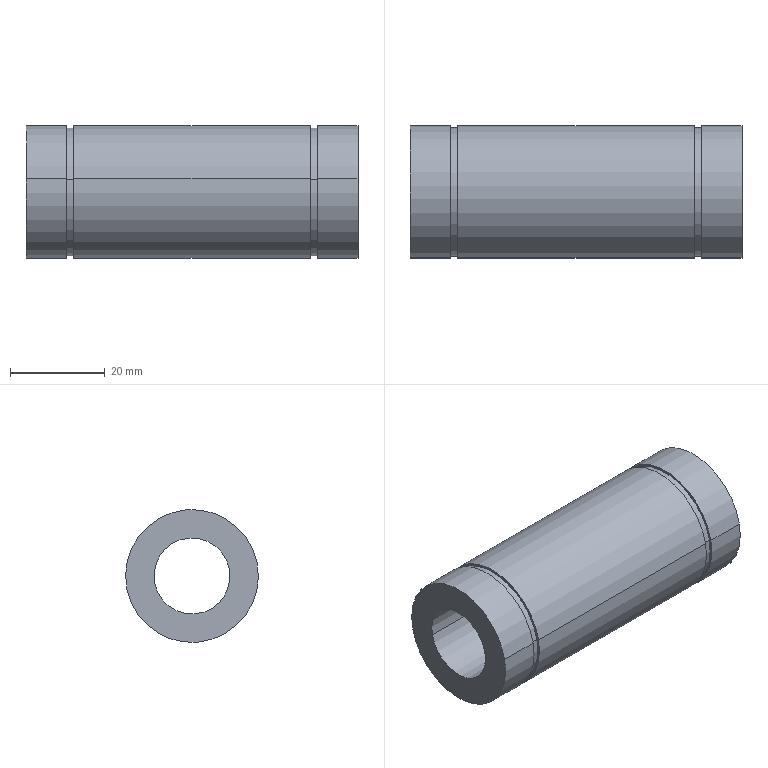Component | SolidWorks | DoubleFilmTransport-1_BearingLM16LUU-1 | 1 solid | 18 faces | box 70 x 28 x 28 mm | volume 28890 mm3 | cylinder 12 | plane 6 | commonest cylinder face diameters 28 x6 27 x4 16 x2
STEP:
#1=CARTESIAN_POINT('',(-7.398,6.758,0.6412));
#2=VERTEX_POINT('',#1);
#3=CARTESIAN_POINT('',(-7.398,7.838,0.4218));
#4=VERTEX_POINT('',#3);
#5=CARTESIAN_POINT('',(-7.398,7.298,0.5315));
#6=DIRECTION('',(-1.,0.,0.));
#7=DIRECTION('',(0.,-0.98,0.1991));
#8=AXIS2_PLACEMENT_3D('',#5,#6,#7);
#9=CIRCLE('',#8,0.5512);
#10=EDGE_CURVE('',#2,#4,#9,.T.);
#11=ORIENTED_EDGE('',*,*,#10,.T.);
#12=CARTESIAN_POINT('',(-9.359,7.838,0.4218));
#13=VERTEX_POINT('',#12);
#14=CARTESIAN_POINT('',(-9.757,7.838,0.4218));
#15=DIRECTION('',(-1.,0.,0.));
#16=VECTOR('',#15,39.37);
#17=LINE('',#14,#16);
#18=EDGE_CURVE('',#4,#13,#17,.T.);
#19=ORIENTED_EDGE('',*,*,#18,.T.);
#20=CARTESIAN_POINT('',(-9.359,6.758,0.6412));
#21=VERTEX_POINT('',#20);
#22=CARTESIAN_POINT('',(-9.359,7.298,0.5315));
#23=DIRECTION('',(1.,0.,0.));
#24=DIRECTION('',(0.,-0.98,0.1991));
#25=AXIS2_PLACEMENT_3D('',#22,#23,#24);
#26=CIRCLE('',#25,0.5512);
#27=EDGE_CURVE('',#13,#21,#26,.T.);
#28=ORIENTED_EDGE('',*,*,#27,.T.);
#29=CARTESIAN_POINT('',(-9.757,6.758,0.6412));
#30=DIRECTION('',(-1.,0.,0.));
#31=VECTOR('',#30,39.37);
#32=LINE('',#29,#31);
#33=EDGE_CURVE('',#2,#21,#32,.T.);
#34=ORIENTED_EDGE('',*,*,#33,.F.);
#35=EDGE_LOOP('',(#11,#19,#28,#34));
#36=FACE_OUTER_BOUND('',#35,.T.);
#37=CARTESIAN_POINT('',(-9.757,7.298,0.5315));
#38=DIRECTION('',(-1.,0.,0.));
#39=DIRECTION('',(0.,-0.98,0.1991));
#40=AXIS2_PLACEMENT_3D('',#37,#38,#39);
#41=CYLINDRICAL_SURFACE('',#40,0.5512);
#42=ADVANCED_FACE('',(#36),#41,.T.);
#43=CARTESIAN_POINT('',(-9.359,6.777,0.6373));
#44=VERTEX_POINT('',#43);
#45=CARTESIAN_POINT('',(-9.359,7.819,0.4257));
#46=VERTEX_POINT('',#45);
#47=CARTESIAN_POINT('',(-9.359,7.298,0.5315));
#48=DIRECTION('',(-1.,0.,0.));
#49=DIRECTION('',(0.,-0.98,0.1991));
#50=AXIS2_PLACEMENT_3D('',#47,#48,#49);
#51=CIRCLE('',#50,0.5315);
#52=EDGE_CURVE('',#44,#46,#51,.T.);
#53=ORIENTED_EDGE('',*,*,#52,.T.);
#54=CARTESIAN_POINT('',(-9.422,7.819,0.4257));
#55=VERTEX_POINT('',#54);
#56=CARTESIAN_POINT('',(-9.757,7.819,0.4257));
#57=DIRECTION('',(-1.,0.,0.));
#58=VECTOR('',#57,39.37);
#59=LINE('',#56,#58);
#60=EDGE_CURVE('',#46,#55,#59,.T.);
#61=ORIENTED_EDGE('',*,*,#60,.T.);
#62=CARTESIAN_POINT('',(-9.422,6.777,0.6373));
#63=VERTEX_POINT('',#62);
#64=CARTESIAN_POINT('',(-9.422,7.298,0.5315));
#65=DIRECTION('',(1.,0.,0.));
#66=DIRECTION('',(0.,-0.98,0.1991));
#67=AXIS2_PLACEMENT_3D('',#64,#65,#66);
#68=CIRCLE('',#67,0.5315);
#69=EDGE_CURVE('',#55,#63,#68,.T.);
#70=ORIENTED_EDGE('',*,*,#69,.T.);
#71=CARTESIAN_POINT('',(-9.757,6.777,0.6373));
#72=DIRECTION('',(-1.,0.,0.));
#73=VECTOR('',#72,39.37);
#74=LINE('',#71,#73);
#75=EDGE_CURVE('',#44,#63,#74,.T.);
#76=ORIENTED_EDGE('',*,*,#75,.F.);
#77=EDGE_LOOP('',(#53,#61,#70,#76));
#78=FACE_OUTER_BOUND('',#77,.T.);
#79=CARTESIAN_POINT('',(-9.757,7.298,0.5315));
#80=DIRECTION('',(-1.,0.,0.));
#81=DIRECTION('',(0.,-0.98,0.1991));
#82=AXIS2_PLACEMENT_3D('',#79,#80,#81);
#83=CYLINDRICAL_SURFACE('',#82,0.5315);
#84=ADVANCED_FACE('',(#78),#83,.T.);
#85=CARTESIAN_POINT('',(-7.335,6.777,0.6373));
#86=VERTEX_POINT('',#85);
#87=CARTESIAN_POINT('',(-7.335,7.819,0.4257));
#88=VERTEX_POINT('',#87);
#89=CARTESIAN_POINT('',(-7.335,7.298,0.5315));
#90=DIRECTION('',(-1.,0.,0.));
#91=DIRECTION('',(0.,-0.98,0.1991));
#92=AXIS2_PLACEMENT_3D('',#89,#90,#91);
#93=CIRCLE('',#92,0.5315);
#94=EDGE_CURVE('',#86,#88,#93,.T.);
#95=ORIENTED_EDGE('',*,*,#94,.T.);
#96=CARTESIAN_POINT('',(-7.398,7.819,0.4257));
#97=VERTEX_POINT('',#96);
#98=CARTESIAN_POINT('',(-9.757,7.819,0.4257));
#99=DIRECTION('',(-1.,0.,0.));
#100=VECTOR('',#99,39.37);
#101=LINE('',#98,#100);
#102=EDGE_CURVE('',#88,#97,#101,.T.);
#103=ORIENTED_EDGE('',*,*,#102,.T.);
#104=CARTESIAN_POINT('',(-7.398,6.777,0.6373));
#105=VERTEX_POINT('',#104);
#106=CARTESIAN_POINT('',(-7.398,7.298,0.5315));
#107=DIRECTION('',(1.,0.,0.));
#108=DIRECTION('',(0.,-0.98,0.1991));
#109=AXIS2_PLACEMENT_3D('',#106,#107,#108);
#110=CIRCLE('',#109,0.5315);
#111=EDGE_CURVE('',#97,#105,#110,.T.);
#112=ORIENTED_EDGE('',*,*,#111,.T.);
#113=CARTESIAN_POINT('',(-9.757,6.777,0.6373));
#114=DIRECTION('',(-1.,0.,0.));
#115=VECTOR('',#114,39.37);
#116=LINE('',#113,#115);
#117=EDGE_CURVE('',#86,#105,#116,.T.);
#118=ORIENTED_EDGE('',*,*,#117,.F.);
#119=EDGE_LOOP('',(#95,#103,#112,#118));
#120=FACE_OUTER_BOUND('',#119,.T.);
#121=CARTESIAN_POINT('',(-9.757,7.298,0.5315));
#122=DIRECTION('',(-1.,0.,0.));
#123=DIRECTION('',(0.,-0.98,0.1991));
#124=AXIS2_PLACEMENT_3D('',#121,#122,#123);
#125=CYLINDRICAL_SURFACE('',#124,0.5315);
#126=ADVANCED_FACE('',(#120),#125,.T.);
#127=CARTESIAN_POINT('',(-9.422,6.758,0.6412));
#128=VERTEX_POINT('',#127);
#129=CARTESIAN_POINT('',(-9.422,7.838,0.4218));
#130=VERTEX_POINT('',#129);
#131=CARTESIAN_POINT('',(-9.422,7.298,0.5315));
#132=DIRECTION('',(-1.,0.,0.));
#133=DIRECTION('',(0.,-0.98,0.1991));
#134=AXIS2_PLACEMENT_3D('',#131,#132,#133);
#135=CIRCLE('',#134,0.5512);
#136=EDGE_CURVE('',#128,#130,#135,.T.);
#137=ORIENTED_EDGE('',*,*,#136,.T.);
#138=CARTESIAN_POINT('',(-9.757,7.838,0.4218));
#139=VERTEX_POINT('',#138);
#140=CARTESIAN_POINT('',(-9.757,7.838,0.4218));
#141=DIRECTION('',(-1.,0.,0.));
#142=VECTOR('',#141,39.37);
#143=LINE('',#140,#142);
#144=EDGE_CURVE('',#130,#139,#143,.T.);
#145=ORIENTED_EDGE('',*,*,#144,.T.);
#146=CARTESIAN_POINT('',(-9.757,6.758,0.6412));
#147=VERTEX_POINT('',#146);
#148=CARTESIAN_POINT('',(-9.757,7.298,0.5315));
#149=DIRECTION('',(1.,0.,0.));
#150=DIRECTION('',(0.,-0.98,0.1991));
#151=AXIS2_PLACEMENT_3D('',#148,#149,#150);
#152=CIRCLE('',#151,0.5512);
#153=EDGE_CURVE('',#139,#147,#152,.T.);
#154=ORIENTED_EDGE('',*,*,#153,.T.);
#155=CARTESIAN_POINT('',(-9.757,6.758,0.6412));
#156=DIRECTION('',(-1.,0.,0.));
#157=VECTOR('',#156,39.37);
#158=LINE('',#155,#157);
#159=EDGE_CURVE('',#128,#147,#158,.T.);
#160=ORIENTED_EDGE('',*,*,#159,.F.);
#161=EDGE_LOOP('',(#137,#145,#154,#160));
#162=FACE_OUTER_BOUND('',#161,.T.);
#163=CARTESIAN_POINT('',(-9.757,7.298,0.5315));
#164=DIRECTION('',(-1.,0.,0.));
#165=DIRECTION('',(0.,-0.98,0.1991));
#166=AXIS2_PLACEMENT_3D('',#163,#164,#165);
#167=CYLINDRICAL_SURFACE('',#166,0.5512);
#168=ADVANCED_FACE('',(#162),#167,.T.);
#169=CARTESIAN_POINT('',(-7.001,6.758,0.6412));
#170=VERTEX_POINT('',#169);
#171=CARTESIAN_POINT('',(-7.001,7.838,0.4218));
#172=VERTEX_POINT('',#171);
#173=CARTESIAN_POINT('',(-7.001,7.298,0.5315));
#174=DIRECTION('',(-1.,0.,0.));
#175=DIRECTION('',(0.,-0.98,0.1991));
#176=AXIS2_PLACEMENT_3D('',#173,#174,#175);
#177=CIRCLE('',#176,0.5512);
#178=EDGE_CURVE('',#170,#172,#177,.T.);
#179=ORIENTED_EDGE('',*,*,#178,.T.);
#180=CARTESIAN_POINT('',(-7.335,7.838,0.4218));
#181=VERTEX_POINT('',#180);
#182=CARTESIAN_POINT('',(-9.757,7.838,0.4218));
#183=DIRECTION('',(-1.,0.,0.));
#184=VECTOR('',#183,39.37);
#185=LINE('',#182,#184);
#186=EDGE_CURVE('',#172,#181,#185,.T.);
#187=ORIENTED_EDGE('',*,*,#186,.T.);
#188=CARTESIAN_POINT('',(-7.335,6.758,0.6412));
#189=VERTEX_POINT('',#188);
#190=CARTESIAN_POINT('',(-7.335,7.298,0.5315));
#191=DIRECTION('',(1.,0.,0.));
#192=DIRECTION('',(0.,-0.98,0.1991));
#193=AXIS2_PLACEMENT_3D('',#190,#191,#192);
#194=CIRCLE('',#193,0.5512);
#195=EDGE_CURVE('',#181,#189,#194,.T.);
#196=ORIENTED_EDGE('',*,*,#195,.T.);
#197=CARTESIAN_POINT('',(-9.757,6.758,0.6412));
#198=DIRECTION('',(-1.,0.,0.));
#199=VECTOR('',#198,39.37);
#200=LINE('',#197,#199);
#201=EDGE_CURVE('',#170,#189,#200,.T.);
#202=ORIENTED_EDGE('',*,*,#201,.F.);
#203=EDGE_LOOP('',(#179,#187,#196,#202));
#204=FACE_OUTER_BOUND('',#203,.T.);
#205=CARTESIAN_POINT('',(-9.757,7.298,0.5315));
#206=DIRECTION('',(-1.,0.,0.));
#207=DIRECTION('',(0.,-0.98,0.1991));
#208=AXIS2_PLACEMENT_3D('',#205,#206,#207);
#209=CYLINDRICAL_SURFACE('',#208,0.5512);
#210=ADVANCED_FACE('',(#204),#209,.T.);
#211=CARTESIAN_POINT('',(-7.001,6.99,0.5942));
#212=VERTEX_POINT('',#211);
#213=CARTESIAN_POINT('',(-7.001,7.607,0.4688));
#214=VERTEX_POINT('',#213);
#215=CARTESIAN_POINT('',(-7.001,7.298,0.5315));
#216=DIRECTION('',(1.,0.,0.));
#217=DIRECTION('',(0.,-0.98,0.1991));
#218=AXIS2_PLACEMENT_3D('',#215,#216,#217);
#219=CIRCLE('',#218,0.315);
#220=EDGE_CURVE('',#212,#214,#219,.T.);
#221=ORIENTED_EDGE('',*,*,#220,.T.);
#222=CARTESIAN_POINT('',(-9.757,7.607,0.4688));
#223=VERTEX_POINT('',#222);
#224=CARTESIAN_POINT('',(-9.757,7.607,0.4688));
#225=DIRECTION('',(-1.,0.,0.));
#226=VECTOR('',#225,39.37);
#227=LINE('',#224,#226);
#228=EDGE_CURVE('',#214,#223,#227,.T.);
#229=ORIENTED_EDGE('',*,*,#228,.T.);
#230=CARTESIAN_POINT('',(-9.757,6.99,0.5942));
#231=VERTEX_POINT('',#230);
#232=CARTESIAN_POINT('',(-9.757,7.298,0.5315));
#233=DIRECTION('',(-1.,0.,0.));
#234=DIRECTION('',(0.,-0.98,0.1991));
#235=AXIS2_PLACEMENT_3D('',#232,#233,#234);
#236=CIRCLE('',#235,0.315);
#237=EDGE_CURVE('',#223,#231,#236,.T.);
#238=ORIENTED_EDGE('',*,*,#237,.T.);
#239=CARTESIAN_POINT('',(-9.757,6.99,0.5942));
#240=DIRECTION('',(-1.,0.,0.));
#241=VECTOR('',#240,39.37);
#242=LINE('',#239,#241);
#243=EDGE_CURVE('',#212,#231,#242,.T.);
#244=ORIENTED_EDGE('',*,*,#243,.F.);
#245=EDGE_LOOP('',(#221,#229,#238,#244));
#246=FACE_OUTER_BOUND('',#245,.T.);
#247=CARTESIAN_POINT('',(-9.757,7.298,0.5315));
#248=DIRECTION('',(-1.,0.,0.));
#249=DIRECTION('',(0.,-0.98,0.1991));
#250=AXIS2_PLACEMENT_3D('',#247,#248,#249);
#251=CYLINDRICAL_SURFACE('',#250,0.315);
#252=ADVANCED_FACE('',(#246),#251,.F.);
#253=ORIENTED_EDGE('',*,*,#18,.F.);
#254=CARTESIAN_POINT('',(-7.398,7.298,0.5315));
#255=DIRECTION('',(-1.,0.,0.));
#256=DIRECTION('',(0.,-0.98,0.1991));
#257=AXIS2_PLACEMENT_3D('',#254,#255,#256);
#258=CIRCLE('',#257,0.5512);
#259=EDGE_CURVE('',#4,#2,#258,.T.);
#260=ORIENTED_EDGE('',*,*,#259,.T.);
#261=ORIENTED_EDGE('',*,*,#33,.T.);
#262=CARTESIAN_POINT('',(-9.359,7.298,0.5315));
#263=DIRECTION('',(1.,0.,0.));
#264=DIRECTION('',(0.,-0.98,0.1991));
#265=AXIS2_PLACEMENT_3D('',#262,#263,#264);
#266=CIRCLE('',#265,0.5512);
#267=EDGE_CURVE('',#21,#13,#266,.T.);
#268=ORIENTED_EDGE('',*,*,#267,.T.);
#269=EDGE_LOOP('',(#253,#260,#261,#268));
#270=FACE_OUTER_BOUND('',#269,.T.);
#271=CARTESIAN_POINT('',(-9.757,7.298,0.5315));
#272=DIRECTION('',(-1.,0.,0.));
#273=DIRECTION('',(0.,-0.98,0.1991));
#274=AXIS2_PLACEMENT_3D('',#271,#272,#273);
#275=CYLINDRICAL_SURFACE('',#274,0.5512);
#276=ADVANCED_FACE('',(#270),#275,.T.);
#277=ORIENTED_EDGE('',*,*,#52,.F.);
#278=CARTESIAN_POINT('',(-9.359,7.298,0.5315));
#279=DIRECTION('',(-1.,0.,0.));
#280=DIRECTION('',(0.,-0.98,0.1991));
#281=AXIS2_PLACEMENT_3D('',#278,#279,#280);
#282=CIRCLE('',#281,0.5315);
#283=EDGE_CURVE('',#46,#44,#282,.T.);
#284=ORIENTED_EDGE('',*,*,#283,.F.);
#285=EDGE_LOOP('',(#277,#284));
#286=FACE_BOUND('',#285,.T.);
#287=ORIENTED_EDGE('',*,*,#267,.F.);
#288=ORIENTED_EDGE('',*,*,#27,.F.);
#289=EDGE_LOOP('',(#287,#288));
#290=FACE_OUTER_BOUND('',#289,.T.);
#291=CARTESIAN_POINT('',(-9.359,7.408,1.072));
#292=DIRECTION('',(1.,0.,0.));
#293=DIRECTION('',(0.,0.98,-0.1991));
#294=AXIS2_PLACEMENT_3D('',#291,#292,#293);
#295=PLANE('',#294);
#296=ADVANCED_FACE('',(#286,#290),#295,.F.);
#297=ORIENTED_EDGE('',*,*,#10,.F.);
#298=ORIENTED_EDGE('',*,*,#259,.F.);
#299=EDGE_LOOP('',(#297,#298));
#300=FACE_OUTER_BOUND('',#299,.T.);
#301=CARTESIAN_POINT('',(-7.398,7.298,0.5315));
#302=DIRECTION('',(1.,0.,0.));
#303=DIRECTION('',(0.,-0.98,0.1991));
#304=AXIS2_PLACEMENT_3D('',#301,#302,#303);
#305=CIRCLE('',#304,0.5315);
#306=EDGE_CURVE('',#105,#97,#305,.T.);
#307=ORIENTED_EDGE('',*,*,#306,.F.);
#308=ORIENTED_EDGE('',*,*,#111,.F.);
#309=EDGE_LOOP('',(#307,#308));
#310=FACE_BOUND('',#309,.T.);
#311=CARTESIAN_POINT('',(-7.398,7.404,1.052));
#312=DIRECTION('',(-1.,0.,0.));
#313=DIRECTION('',(0.,-0.98,0.1991));
#314=AXIS2_PLACEMENT_3D('',#311,#312,#313);
#315=PLANE('',#314);
#316=ADVANCED_FACE('',(#300,#310),#315,.F.);
#317=ORIENTED_EDGE('',*,*,#60,.F.);
#318=ORIENTED_EDGE('',*,*,#283,.T.);
#319=ORIENTED_EDGE('',*,*,#75,.T.);
#320=CARTESIAN_POINT('',(-9.422,7.298,0.5315));
#321=DIRECTION('',(1.,0.,0.));
#322=DIRECTION('',(0.,-0.98,0.1991));
#323=AXIS2_PLACEMENT_3D('',#320,#321,#322);
#324=CIRCLE('',#323,0.5315);
#325=EDGE_CURVE('',#63,#55,#324,.T.);
#326=ORIENTED_EDGE('',*,*,#325,.T.);
#327=EDGE_LOOP('',(#317,#318,#319,#326));
#328=FACE_OUTER_BOUND('',#327,.T.);
#329=CARTESIAN_POINT('',(-9.757,7.298,0.5315));
#330=DIRECTION('',(-1.,0.,0.));
#331=DIRECTION('',(0.,-0.98,0.1991));
#332=AXIS2_PLACEMENT_3D('',#329,#330,#331);
#333=CYLINDRICAL_SURFACE('',#332,0.5315);
#334=ADVANCED_FACE('',(#328),#333,.T.);
#335=ORIENTED_EDGE('',*,*,#102,.F.);
#336=CARTESIAN_POINT('',(-7.335,7.298,0.5315));
#337=DIRECTION('',(-1.,0.,0.));
#338=DIRECTION('',(0.,-0.98,0.1991));
#339=AXIS2_PLACEMENT_3D('',#336,#337,#338);
#340=CIRCLE('',#339,0.5315);
#341=EDGE_CURVE('',#88,#86,#340,.T.);
#342=ORIENTED_EDGE('',*,*,#341,.T.);
#343=ORIENTED_EDGE('',*,*,#117,.T.);
#344=ORIENTED_EDGE('',*,*,#306,.T.);
#345=EDGE_LOOP('',(#335,#342,#343,#344));
#346=FACE_OUTER_BOUND('',#345,.T.);
#347=CARTESIAN_POINT('',(-9.757,7.298,0.5315));
#348=DIRECTION('',(-1.,0.,0.));
#349=DIRECTION('',(0.,-0.98,0.1991));
#350=AXIS2_PLACEMENT_3D('',#347,#348,#349);
#351=CYLINDRICAL_SURFACE('',#350,0.5315);
#352=ADVANCED_FACE('',(#346),#351,.T.);
#353=ORIENTED_EDGE('',*,*,#136,.F.);
#354=CARTESIAN_POINT('',(-9.422,7.298,0.5315));
#355=DIRECTION('',(-1.,0.,0.));
#356=DIRECTION('',(0.,-0.98,0.1991));
#357=AXIS2_PLACEMENT_3D('',#354,#355,#356);
#358=CIRCLE('',#357,0.5512);
#359=EDGE_CURVE('',#130,#128,#358,.T.);
#360=ORIENTED_EDGE('',*,*,#359,.F.);
#361=EDGE_LOOP('',(#353,#360));
#362=FACE_OUTER_BOUND('',#361,.T.);
#363=ORIENTED_EDGE('',*,*,#325,.F.);
#364=ORIENTED_EDGE('',*,*,#69,.F.);
#365=EDGE_LOOP('',(#363,#364));
#366=FACE_BOUND('',#365,.T.);
#367=CARTESIAN_POINT('',(-9.422,7.404,1.052));
#368=DIRECTION('',(-1.,0.,0.));
#369=DIRECTION('',(0.,-0.98,0.1991));
#370=AXIS2_PLACEMENT_3D('',#367,#368,#369);
#371=PLANE('',#370);
#372=ADVANCED_FACE('',(#362,#366),#371,.F.);
#373=ORIENTED_EDGE('',*,*,#94,.F.);
#374=ORIENTED_EDGE('',*,*,#341,.F.);
#375=EDGE_LOOP('',(#373,#374));
#376=FACE_BOUND('',#375,.T.);
#377=CARTESIAN_POINT('',(-7.335,7.298,0.5315));
#378=DIRECTION('',(1.,0.,0.));
#379=DIRECTION('',(0.,-0.98,0.1991));
#380=AXIS2_PLACEMENT_3D('',#377,#378,#379);
#381=CIRCLE('',#380,0.5512);
#382=EDGE_CURVE('',#189,#181,#381,.T.);
#383=ORIENTED_EDGE('',*,*,#382,.F.);
#384=ORIENTED_EDGE('',*,*,#195,.F.);
#385=EDGE_LOOP('',(#383,#384));
#386=FACE_OUTER_BOUND('',#385,.T.);
#387=CARTESIAN_POINT('',(-7.335,7.404,1.052));
#388=DIRECTION('',(1.,0.,0.));
#389=DIRECTION('',(0.,0.98,-0.1991));
#390=AXIS2_PLACEMENT_3D('',#387,#388,#389);
#391=PLANE('',#390);
#392=ADVANCED_FACE('',(#376,#386),#391,.F.);
#393=ORIENTED_EDGE('',*,*,#144,.F.);
#394=ORIENTED_EDGE('',*,*,#359,.T.);
#395=ORIENTED_EDGE('',*,*,#159,.T.);
#396=CARTESIAN_POINT('',(-9.757,7.298,0.5315));
#397=DIRECTION('',(1.,0.,0.));
#398=DIRECTION('',(0.,-0.98,0.1991));
#399=AXIS2_PLACEMENT_3D('',#396,#397,#398);
#400=CIRCLE('',#399,0.5512);
#401=EDGE_CURVE('',#147,#139,#400,.T.);
#402=ORIENTED_EDGE('',*,*,#401,.T.);
#403=EDGE_LOOP('',(#393,#394,#395,#402));
#404=FACE_OUTER_BOUND('',#403,.T.);
#405=CARTESIAN_POINT('',(-9.757,7.298,0.5315));
#406=DIRECTION('',(-1.,0.,0.));
#407=DIRECTION('',(0.,-0.98,0.1991));
#408=AXIS2_PLACEMENT_3D('',#405,#406,#407);
#409=CYLINDRICAL_SURFACE('',#408,0.5512);
#410=ADVANCED_FACE('',(#404),#409,.T.);
#411=ORIENTED_EDGE('',*,*,#186,.F.);
#412=CARTESIAN_POINT('',(-7.001,7.298,0.5315));
#413=DIRECTION('',(-1.,0.,0.));
#414=DIRECTION('',(0.,-0.98,0.1991));
#415=AXIS2_PLACEMENT_3D('',#412,#413,#414);
#416=CIRCLE('',#415,0.5512);
#417=EDGE_CURVE('',#172,#170,#416,.T.);
#418=ORIENTED_EDGE('',*,*,#417,.T.);
#419=ORIENTED_EDGE('',*,*,#201,.T.);
#420=ORIENTED_EDGE('',*,*,#382,.T.);
#421=EDGE_LOOP('',(#411,#418,#419,#420));
#422=FACE_OUTER_BOUND('',#421,.T.);
#423=CARTESIAN_POINT('',(-9.757,7.298,0.5315));
#424=DIRECTION('',(-1.,0.,0.));
#425=DIRECTION('',(0.,-0.98,0.1991));
#426=AXIS2_PLACEMENT_3D('',#423,#424,#425);
#427=CYLINDRICAL_SURFACE('',#426,0.5512);
#428=ADVANCED_FACE('',(#422),#427,.T.);
#429=CARTESIAN_POINT('',(-9.757,7.298,0.5315));
#430=DIRECTION('',(-1.,0.,0.));
#431=DIRECTION('',(0.,-0.98,0.1991));
#432=AXIS2_PLACEMENT_3D('',#429,#430,#431);
#433=CIRCLE('',#432,0.315);
#434=EDGE_CURVE('',#231,#223,#433,.T.);
#435=ORIENTED_EDGE('',*,*,#434,.F.);
#436=ORIENTED_EDGE('',*,*,#237,.F.);
#437=EDGE_LOOP('',(#435,#436));
#438=FACE_BOUND('',#437,.T.);
#439=ORIENTED_EDGE('',*,*,#401,.F.);
#440=ORIENTED_EDGE('',*,*,#153,.F.);
#441=EDGE_LOOP('',(#439,#440));
#442=FACE_OUTER_BOUND('',#441,.T.);
#443=CARTESIAN_POINT('',(-9.757,7.408,1.072));
#444=DIRECTION('',(1.,0.,0.));
#445=DIRECTION('',(0.,0.98,-0.1991));
#446=AXIS2_PLACEMENT_3D('',#443,#444,#445);
#447=PLANE('',#446);
#448=ADVANCED_FACE('',(#438,#442),#447,.F.);
#449=ORIENTED_EDGE('',*,*,#178,.F.);
#450=ORIENTED_EDGE('',*,*,#417,.F.);
#451=EDGE_LOOP('',(#449,#450));
#452=FACE_OUTER_BOUND('',#451,.T.);
#453=ORIENTED_EDGE('',*,*,#220,.F.);
#454=CARTESIAN_POINT('',(-7.001,7.298,0.5315));
#455=DIRECTION('',(1.,0.,0.));
#456=DIRECTION('',(0.,-0.98,0.1991));
#457=AXIS2_PLACEMENT_3D('',#454,#455,#456);
#458=CIRCLE('',#457,0.315);
#459=EDGE_CURVE('',#214,#212,#458,.T.);
#460=ORIENTED_EDGE('',*,*,#459,.F.);
#461=EDGE_LOOP('',(#453,#460));
#462=FACE_BOUND('',#461,.T.);
#463=CARTESIAN_POINT('',(-7.001,7.361,0.8402));
#464=DIRECTION('',(-1.,0.,0.));
#465=DIRECTION('',(0.,-0.98,0.1991));
#466=AXIS2_PLACEMENT_3D('',#463,#464,#465);
#467=PLANE('',#466);
#468=ADVANCED_FACE('',(#452,#462),#467,.F.);
#469=ORIENTED_EDGE('',*,*,#228,.F.);
#470=ORIENTED_EDGE('',*,*,#459,.T.);
#471=ORIENTED_EDGE('',*,*,#243,.T.);
#472=ORIENTED_EDGE('',*,*,#434,.T.);
#473=EDGE_LOOP('',(#469,#470,#471,#472));
#474=FACE_OUTER_BOUND('',#473,.T.);
#475=CARTESIAN_POINT('',(-9.757,7.298,0.5315));
#476=DIRECTION('',(-1.,0.,0.));
#477=DIRECTION('',(0.,-0.98,0.1991));
#478=AXIS2_PLACEMENT_3D('',#475,#476,#477);
#479=CYLINDRICAL_SURFACE('',#478,0.315);
#480=ADVANCED_FACE('',(#474),#479,.F.);
#481=CLOSED_SHELL('',(#42,#84,#126,#168,#210,#252,#276,#296,#316,#334,#352,#372,#392,#410,#428,#448,#468,#480));
#482=MANIFOLD_SOLID_BREP('',#481);
#483=CARTESIAN_POINT('',(0.,0.,0.));
#484=DIRECTION('',(0.,0.,1.));
#485=DIRECTION('',(1.,0.,0.));
#486=AXIS2_PLACEMENT_3D('',#483,#484,#485);
#487=(LENGTH_UNIT()NAMED_UNIT(*)SI_UNIT($,.METRE.));
#488=LENGTH_MEASURE_WITH_UNIT(LENGTH_MEASURE(0.0254),#487);
#489=DIMENSIONAL_EXPONENTS(1.,0.,0.,0.,0.,0.,0.);
#490=(CONVERSION_BASED_UNIT('',#488)LENGTH_UNIT()NAMED_UNIT(#489));
#491=UNCERTAINTY_MEASURE_WITH_UNIT(LENGTH_MEASURE(0.00001),#490,'','');
#492=(NAMED_UNIT(*)PLANE_ANGLE_UNIT()SI_UNIT($,.RADIAN.));
#493=(NAMED_UNIT(*)SI_UNIT($,.STERADIAN.)SOLID_ANGLE_UNIT());
#494=(GEOMETRIC_REPRESENTATION_CONTEXT(3)GLOBAL_UNCERTAINTY_ASSIGNED_CONTEXT((#491))GLOBAL_UNIT_ASSIGNED_CONTEXT((#490,#492,#493))REPRESENTATION_CONTEXT('',''));
#495=ADVANCED_BREP_SHAPE_REPRESENTATION('',(#482,#486),#494);
#496=COLOUR_RGB('',0.7922,0.8196,0.9333);
#497=FILL_AREA_STYLE_COLOUR('',#496);
#498=FILL_AREA_STYLE('',(#497));
#499=SURFACE_STYLE_FILL_AREA(#498);
#500=SURFACE_SIDE_STYLE('',(#499));
#501=SURFACE_STYLE_USAGE(.BOTH.,#500);
#502=PRESENTATION_STYLE_ASSIGNMENT((#501));
#503=STYLED_ITEM('',(#502),#482);
#504=(LENGTH_UNIT()NAMED_UNIT(*)SI_UNIT($,.METRE.));
#505=LENGTH_MEASURE_WITH_UNIT(LENGTH_MEASURE(0.0254),#504);
#506=DIMENSIONAL_EXPONENTS(1.,0.,0.,0.,0.,0.,0.);
#507=(CONVERSION_BASED_UNIT('',#505)LENGTH_UNIT()NAMED_UNIT(#506));
#508=UNCERTAINTY_MEASURE_WITH_UNIT(LENGTH_MEASURE(0.00001),#507,'','');
#509=(NAMED_UNIT(*)PLANE_ANGLE_UNIT()SI_UNIT($,.RADIAN.));
#510=(NAMED_UNIT(*)SI_UNIT($,.STERADIAN.)SOLID_ANGLE_UNIT());
#511=(GEOMETRIC_REPRESENTATION_CONTEXT(3)GLOBAL_UNCERTAINTY_ASSIGNED_CONTEXT((#508))GLOBAL_UNIT_ASSIGNED_CONTEXT((#507,#509,#510))REPRESENTATION_CONTEXT('',''));
#512=MECHANICAL_DESIGN_GEOMETRIC_PRESENTATION_REPRESENTATION('',(#503),#511);
#513=PRESENTATION_LAYER_ASSIGNMENT('','',(#503));